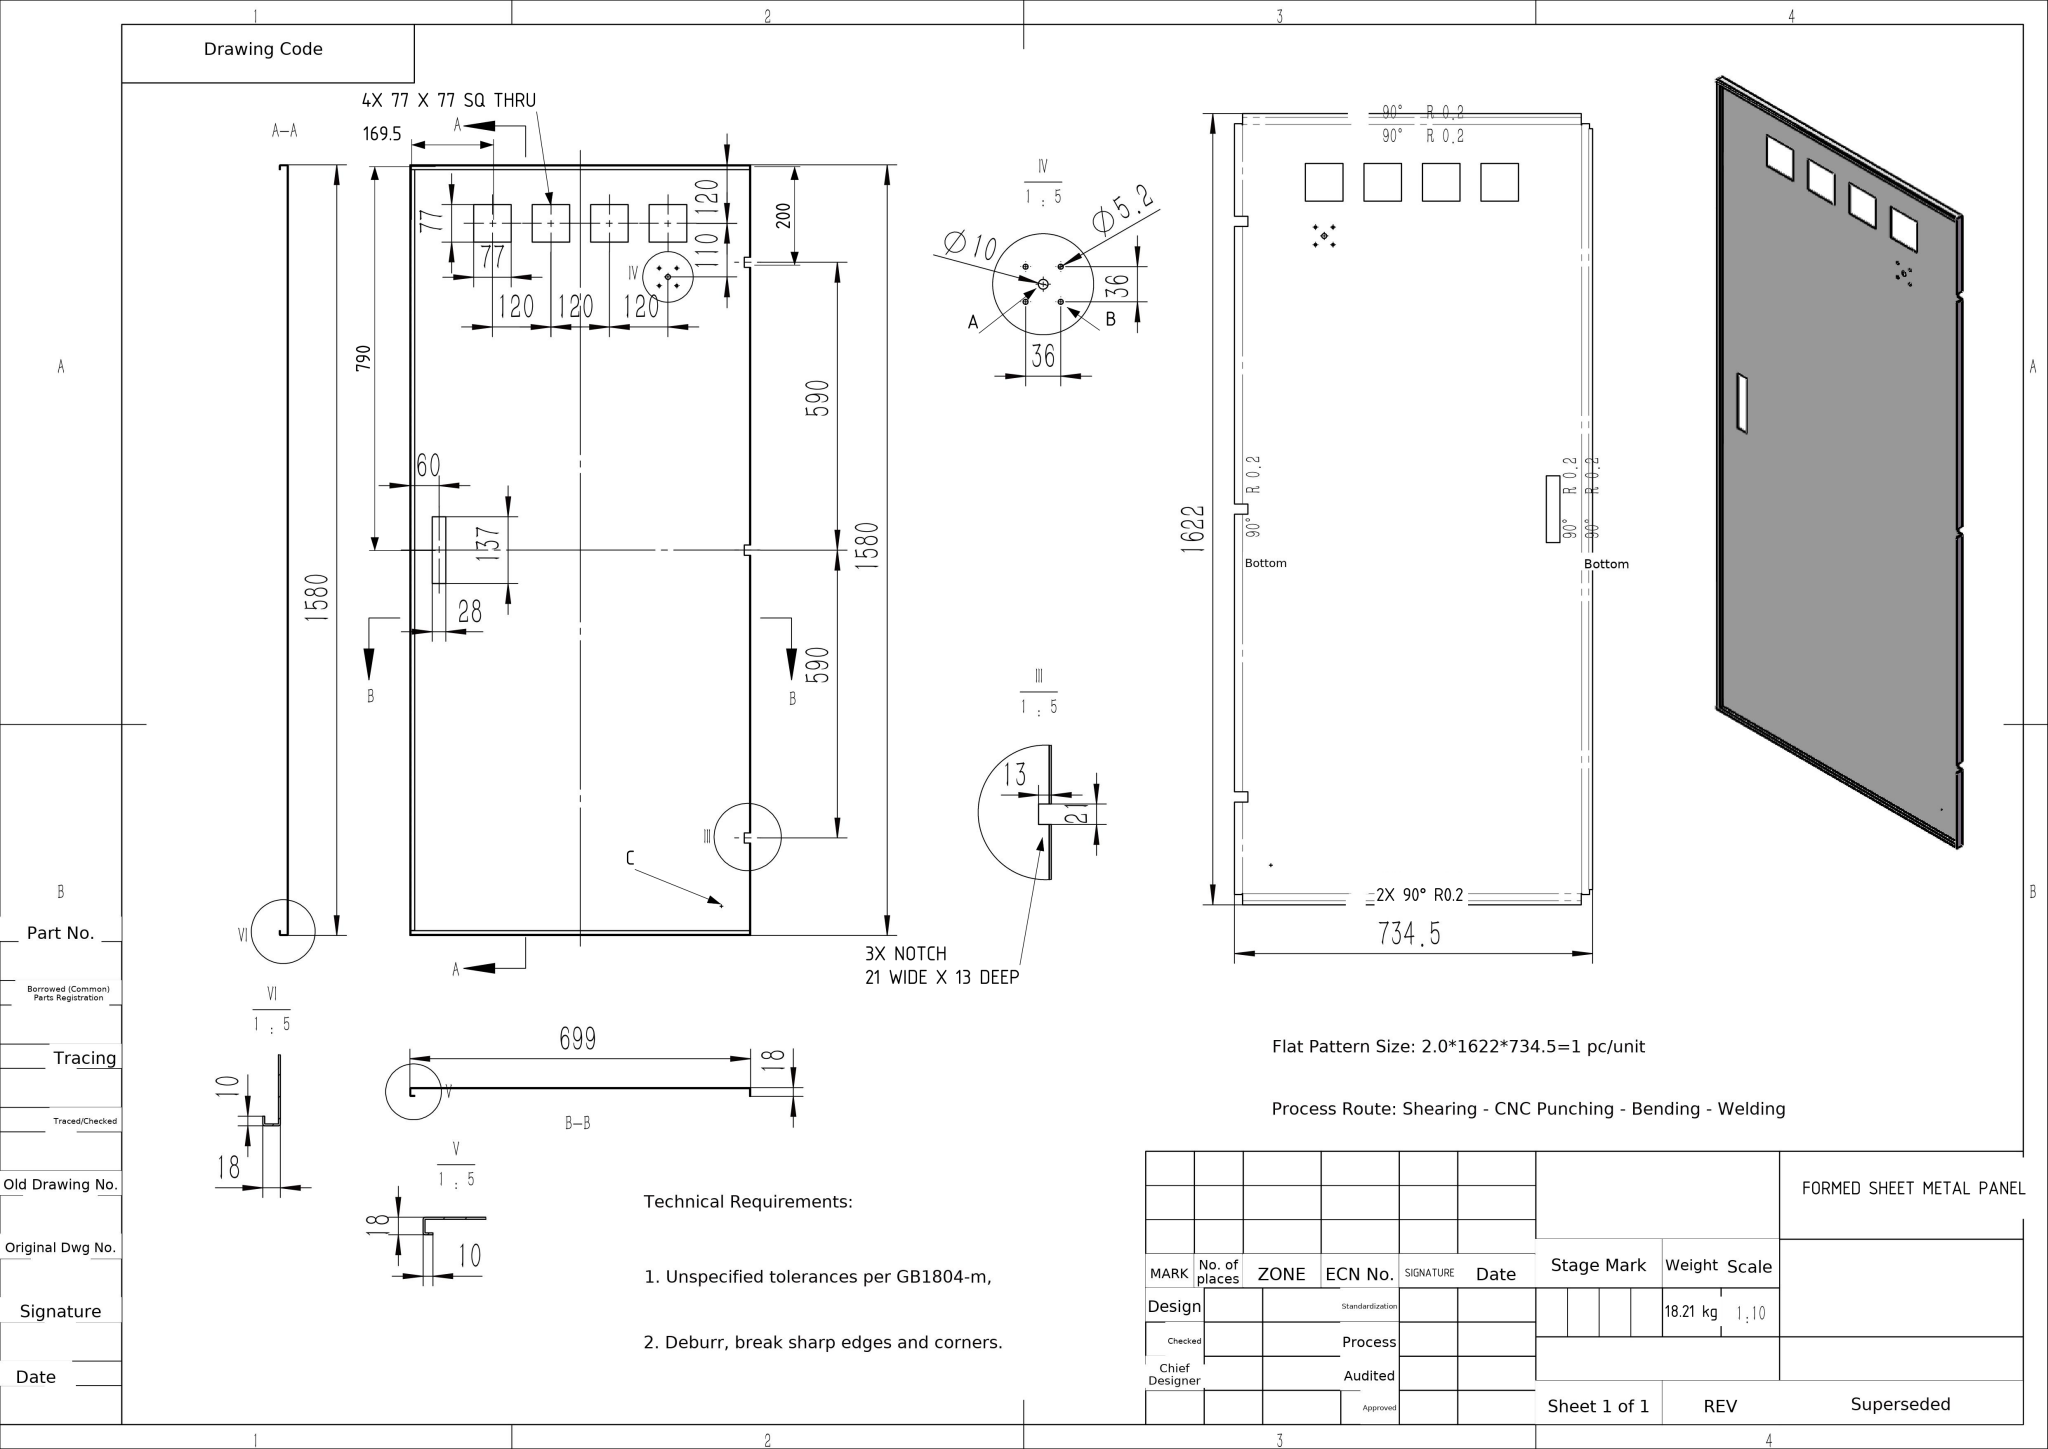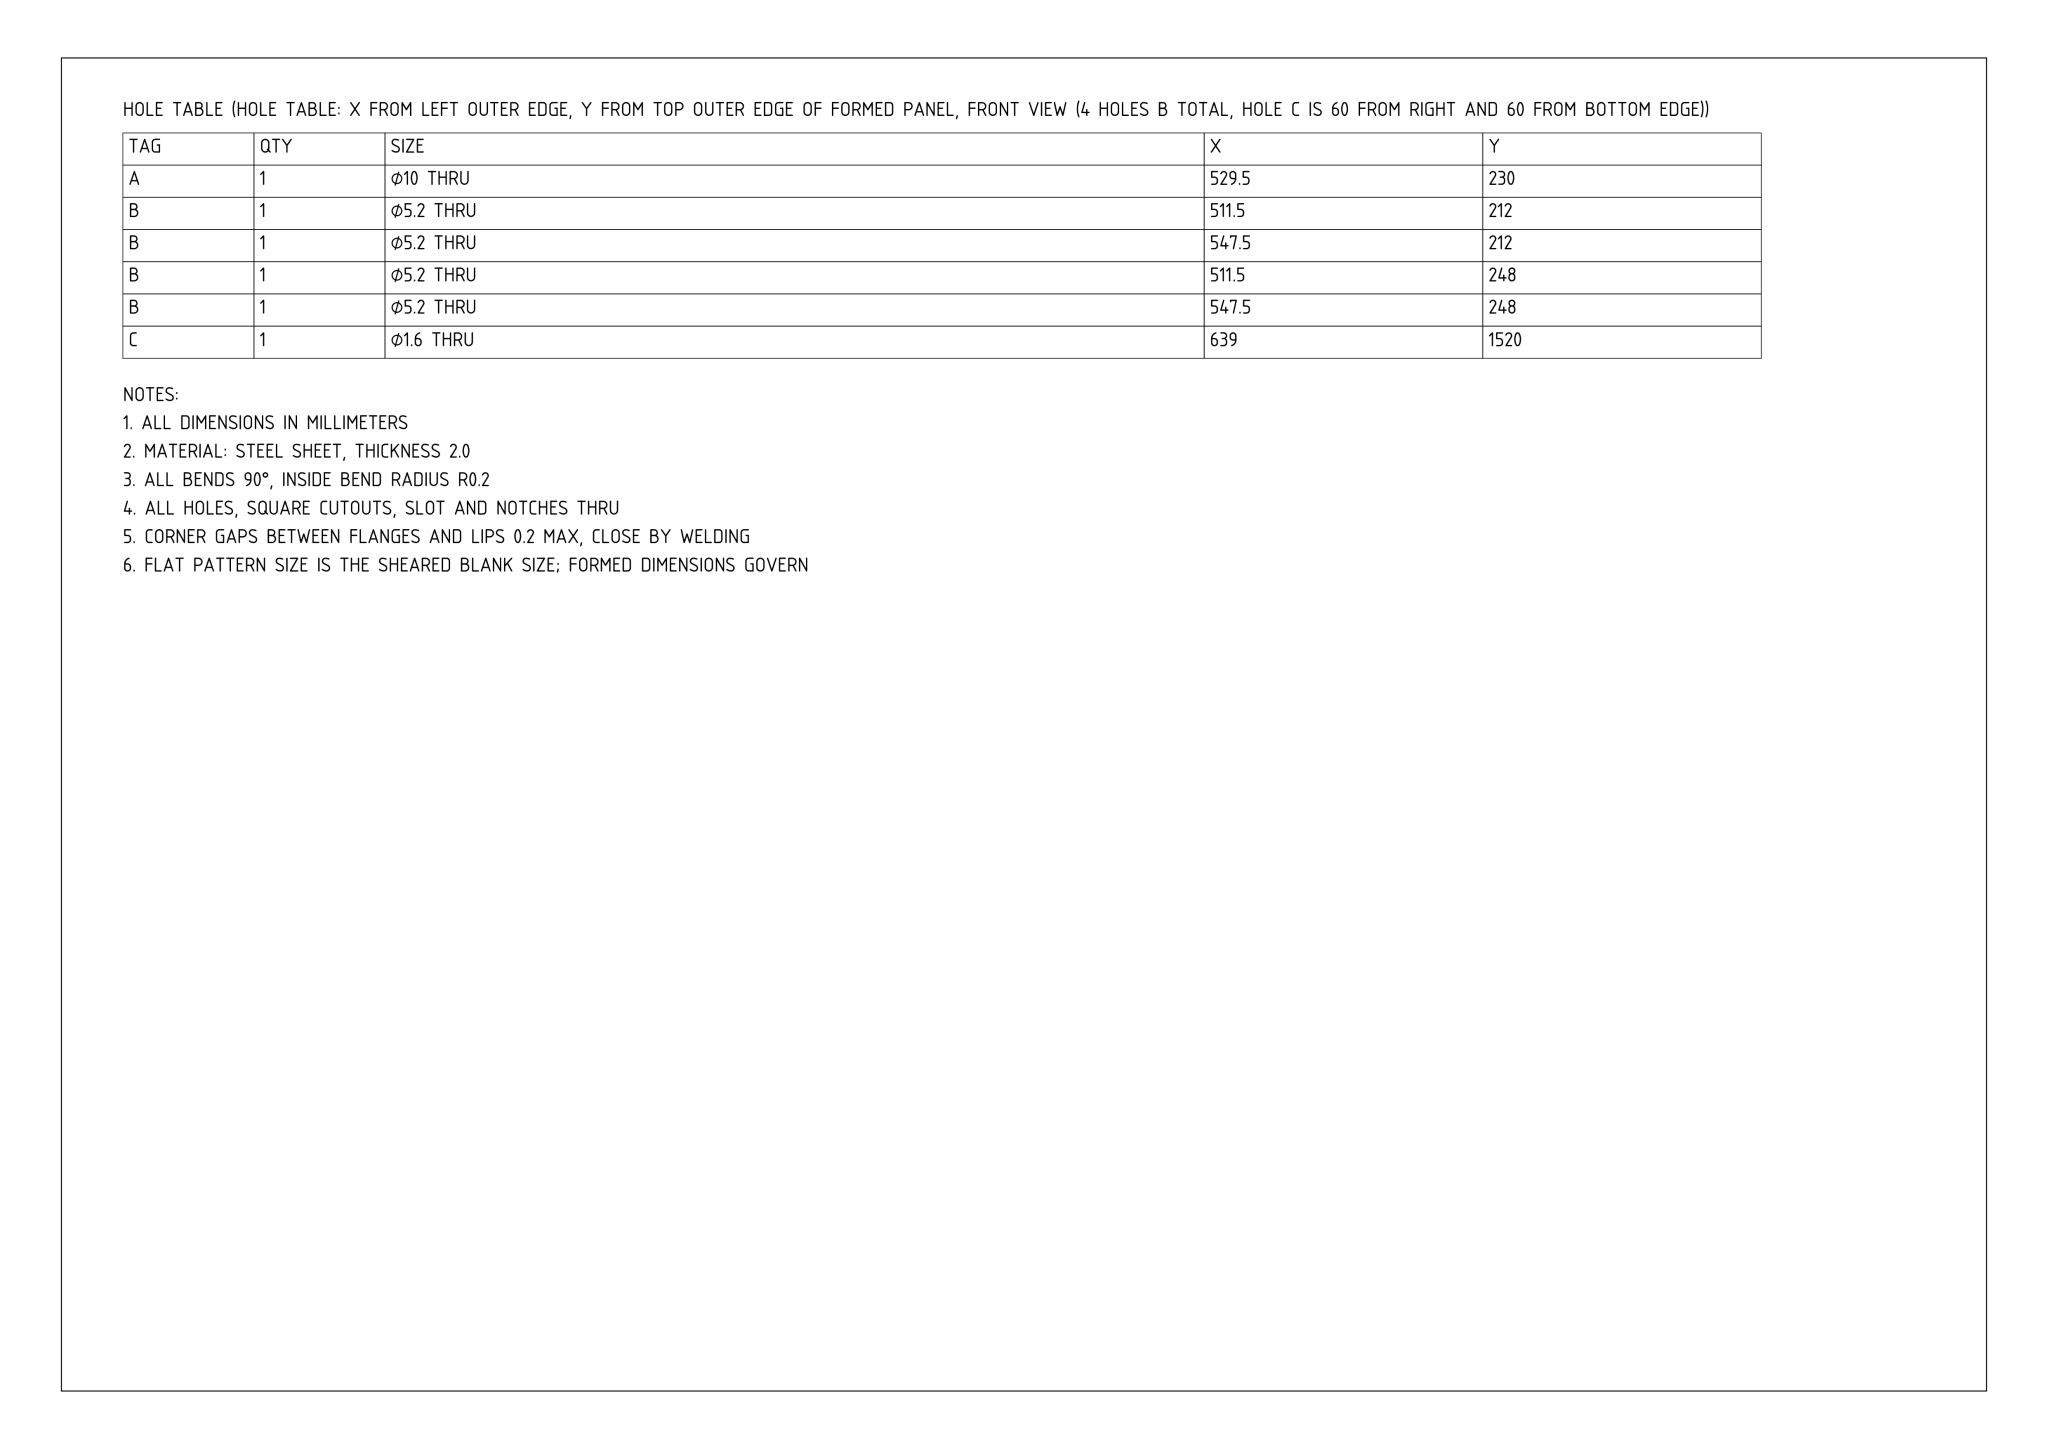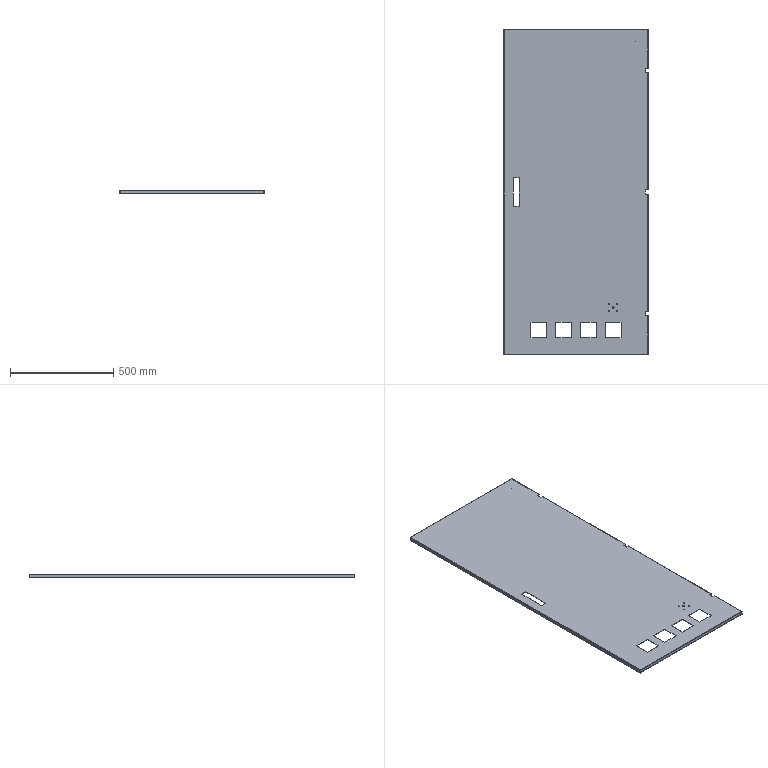Part | NX | mm | 1 solid | 138 faces | box 699 x 1580 x 18 mm | volume 2334814 mm3 | plane 106 | cylinder 32 | commonest cylinder face diameters 4.4 x10 0.4 x10 5.2 x8 10 x2 1.6 x2